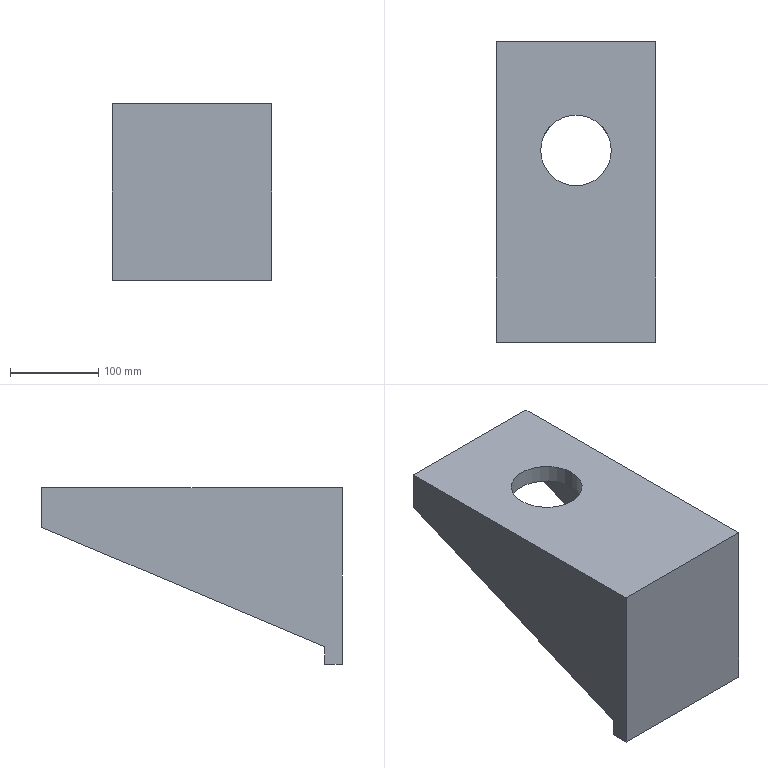Component | SolidWorks | CylinderBaseBaffle-1 | 1 solid | 14 faces | box 180 x 340 x 200 mm | volume 2955469 mm3 | plane 12 | cylinder 2 | commonest cylinder face diameters 80 x2
build123d program:
from build123d import *

# Parameters (mm, degrees)
SKETCH1_W           = 180
SKETCH1_H           = 320
BOSS_EXTRUDE1_DEPTH = 20
SKETCH2_W           = 180
SKETCH2_H           = 200
BOSS_EXTRUDE2_DEPTH = 20
BOSS_EXTRUDE3_DEPTH = 20
SKETCH5_R           = 40
CUT_EXTRUDE2_DEPTH  = 50


with BuildPart() as part:
    # Sketch1 → Boss-Extrude1 (new body)
    with BuildSketch(Plane.XY):
        Rectangle(SKETCH1_W, SKETCH1_H)
    extrude(amount=BOSS_EXTRUDE1_DEPTH)

    # Sketch2 → Boss-Extrude2 (add)
    with BuildSketch(Plane.XZ.offset(160)):
        with Locations((0, -80)):
            Rectangle(SKETCH2_W, SKETCH2_H)
    extrude(amount=BOSS_EXTRUDE2_DEPTH)

    # Sketch3 → Boss-Extrude3 (add)
    with BuildSketch(Plane(origin=(90, 0, 0), x_dir=(0, 0, -1), z_dir=(1, 0, 0))):
        Polygon((0, 160), (25, 160), (160, -160), (0, -160), align=None)
    boss_extrude3 = extrude(amount=-BOSS_EXTRUDE3_DEPTH)

    # Mirror1: Boss-Extrude3 across plane
    add(boss_extrude3.mirror(Plane(origin=(0, 0, 0), x_dir=(0, 0, 1), z_dir=(1, 0, 0))))

    # Sketch5 → Cut-Extrude2 (cut)
    with BuildSketch(Plane(origin=(0, 0, 0), x_dir=(-1, 0, 0), z_dir=(0, 0, -1))):
        with Locations((0, 36.859)):
            Circle(SKETCH5_R)
    extrude(amount=-CUT_EXTRUDE2_DEPTH, mode=Mode.SUBTRACT)


solid = part.part

# Placed as in the assembly
solid = solid.moved(Location((-7.456, -34.275, 560), (0, 0, 0)))
STEP:
#1=COLOUR_RGB('',0.7922,0.8196,0.9333);
#2=FILL_AREA_STYLE_COLOUR('',#1);
#3=FILL_AREA_STYLE('',(#2));
#4=SURFACE_STYLE_FILL_AREA(#3);
#5=SURFACE_SIDE_STYLE('',(#4));
#6=SURFACE_STYLE_USAGE(.BOTH.,#5);
#7=PRESENTATION_STYLE_ASSIGNMENT((#6));
#8=CARTESIAN_POINT('',(-1.868,0.1017,22.835));
#9=VERTEX_POINT('',#8);
#10=CARTESIAN_POINT('',(1.281,0.1017,22.835));
#11=VERTEX_POINT('',#10);
#12=CARTESIAN_POINT('',(-0.2935,0.1017,22.835));
#13=DIRECTION('',(0.,0.,1.));
#14=DIRECTION('',(1.,0.,0.));
#15=AXIS2_PLACEMENT_3D('',#12,#13,#14);
#16=CIRCLE('',#15,1.575);
#17=EDGE_CURVE('',#9,#11,#16,.T.);
#18=ORIENTED_EDGE('',*,*,#17,.T.);
#19=CARTESIAN_POINT('',(1.281,0.1017,22.047));
#20=VERTEX_POINT('',#19);
#21=CARTESIAN_POINT('',(1.281,0.1017,24.016));
#22=DIRECTION('',(0.,0.,-1.));
#23=VECTOR('',#22,39.37);
#24=LINE('',#21,#23);
#25=EDGE_CURVE('',#11,#20,#24,.T.);
#26=ORIENTED_EDGE('',*,*,#25,.T.);
#27=CARTESIAN_POINT('',(-1.868,0.1017,22.047));
#28=VERTEX_POINT('',#27);
#29=CARTESIAN_POINT('',(-0.2935,0.1017,22.047));
#30=DIRECTION('',(0.,0.,-1.));
#31=DIRECTION('',(-1.,0.,0.));
#32=AXIS2_PLACEMENT_3D('',#29,#30,#31);
#33=CIRCLE('',#32,1.575);
#34=EDGE_CURVE('',#20,#28,#33,.T.);
#35=ORIENTED_EDGE('',*,*,#34,.T.);
#36=CARTESIAN_POINT('',(-1.868,0.1017,24.016));
#37=DIRECTION('',(0.,0.,-1.));
#38=VECTOR('',#37,39.37);
#39=LINE('',#36,#38);
#40=EDGE_CURVE('',#9,#28,#39,.T.);
#41=ORIENTED_EDGE('',*,*,#40,.F.);
#42=EDGE_LOOP('',(#18,#26,#35,#41));
#43=FACE_OUTER_BOUND('',#42,.T.);
#44=CARTESIAN_POINT('',(-0.2935,0.1017,24.016));
#45=DIRECTION('',(0.,0.,-1.));
#46=DIRECTION('',(-1.,0.,0.));
#47=AXIS2_PLACEMENT_3D('',#44,#45,#46);
#48=CYLINDRICAL_SURFACE('',#47,1.575);
#49=ADVANCED_FACE('',(#43),#48,.F.);
#50=CARTESIAN_POINT('',(-3.049,-7.649,15.748));
#51=VERTEX_POINT('',#50);
#52=CARTESIAN_POINT('',(-3.837,-7.649,15.748));
#53=VERTEX_POINT('',#52);
#54=CARTESIAN_POINT('',(-3.049,-7.649,15.748));
#55=DIRECTION('',(-1.,0.,0.));
#56=VECTOR('',#55,39.37);
#57=LINE('',#54,#56);
#58=EDGE_CURVE('',#51,#53,#57,.T.);
#59=ORIENTED_EDGE('',*,*,#58,.F.);
#60=CARTESIAN_POINT('',(-3.049,-7.649,22.047));
#61=VERTEX_POINT('',#60);
#62=CARTESIAN_POINT('',(-3.049,-7.649,15.748));
#63=DIRECTION('',(0.,0.,-1.));
#64=VECTOR('',#63,39.37);
#65=LINE('',#62,#64);
#66=EDGE_CURVE('',#61,#51,#65,.T.);
#67=ORIENTED_EDGE('',*,*,#66,.F.);
#68=CARTESIAN_POINT('',(2.462,-7.649,22.047));
#69=VERTEX_POINT('',#68);
#70=CARTESIAN_POINT('',(3.25,-7.649,22.047));
#71=DIRECTION('',(1.,0.,0.));
#72=VECTOR('',#71,39.37);
#73=LINE('',#70,#72);
#74=EDGE_CURVE('',#61,#69,#73,.T.);
#75=ORIENTED_EDGE('',*,*,#74,.T.);
#76=CARTESIAN_POINT('',(2.462,-7.649,15.748));
#77=VERTEX_POINT('',#76);
#78=CARTESIAN_POINT('',(2.462,-7.649,15.748));
#79=DIRECTION('',(0.,0.,-1.));
#80=VECTOR('',#79,39.37);
#81=LINE('',#78,#80);
#82=EDGE_CURVE('',#69,#77,#81,.T.);
#83=ORIENTED_EDGE('',*,*,#82,.T.);
#84=CARTESIAN_POINT('',(3.25,-7.649,15.748));
#85=VERTEX_POINT('',#84);
#86=CARTESIAN_POINT('',(2.462,-7.649,15.748));
#87=DIRECTION('',(1.,0.,0.));
#88=VECTOR('',#87,39.37);
#89=LINE('',#86,#88);
#90=EDGE_CURVE('',#77,#85,#89,.T.);
#91=ORIENTED_EDGE('',*,*,#90,.T.);
#92=CARTESIAN_POINT('',(3.25,-7.649,14.961));
#93=VERTEX_POINT('',#92);
#94=CARTESIAN_POINT('',(3.25,-7.649,22.835));
#95=DIRECTION('',(-0.,0.,1.));
#96=VECTOR('',#95,39.37);
#97=LINE('',#94,#96);
#98=EDGE_CURVE('',#93,#85,#97,.T.);
#99=ORIENTED_EDGE('',*,*,#98,.F.);
#100=CARTESIAN_POINT('',(-3.837,-7.649,14.961));
#101=VERTEX_POINT('',#100);
#102=CARTESIAN_POINT('',(-3.837,-7.649,14.961));
#103=DIRECTION('',(1.,0.,0.));
#104=VECTOR('',#103,39.37);
#105=LINE('',#102,#104);
#106=EDGE_CURVE('',#101,#93,#105,.T.);
#107=ORIENTED_EDGE('',*,*,#106,.F.);
#108=CARTESIAN_POINT('',(-3.837,-7.649,22.835));
#109=DIRECTION('',(0.,0.,-1.));
#110=VECTOR('',#109,39.37);
#111=LINE('',#108,#110);
#112=EDGE_CURVE('',#53,#101,#111,.T.);
#113=ORIENTED_EDGE('',*,*,#112,.F.);
#114=EDGE_LOOP('',(#59,#67,#75,#83,#91,#99,#107,#113));
#115=FACE_OUTER_BOUND('',#114,.T.);
#116=CARTESIAN_POINT('',(-3.837,-7.649,14.961));
#117=DIRECTION('',(0.,-1.,0.));
#118=DIRECTION('',(0.,0.,-1.));
#119=AXIS2_PLACEMENT_3D('',#116,#117,#118);
#120=PLANE('',#119);
#121=ADVANCED_FACE('',(#115),#120,.F.);
#122=CARTESIAN_POINT('',(-3.837,4.95,22.835));
#123=VERTEX_POINT('',#122);
#124=CARTESIAN_POINT('',(-3.837,4.95,21.063));
#125=VERTEX_POINT('',#124);
#126=CARTESIAN_POINT('',(-3.837,4.95,22.835));
#127=DIRECTION('',(0.,0.,-1.));
#128=VECTOR('',#127,39.37);
#129=LINE('',#126,#128);
#130=EDGE_CURVE('',#123,#125,#129,.T.);
#131=ORIENTED_EDGE('',*,*,#130,.T.);
#132=CARTESIAN_POINT('',(-3.837,4.95,21.063));
#133=DIRECTION('',(0.,0.9214,0.3887));
#134=VECTOR('',#133,39.37);
#135=LINE('',#132,#134);
#136=EDGE_CURVE('',#53,#125,#135,.T.);
#137=ORIENTED_EDGE('',*,*,#136,.F.);
#138=ORIENTED_EDGE('',*,*,#112,.T.);
#139=CARTESIAN_POINT('',(-3.837,-8.436,14.961));
#140=VERTEX_POINT('',#139);
#141=CARTESIAN_POINT('',(-3.837,-8.436,14.961));
#142=DIRECTION('',(0.,1.,0.));
#143=VECTOR('',#142,39.37);
#144=LINE('',#141,#143);
#145=EDGE_CURVE('',#140,#101,#144,.T.);
#146=ORIENTED_EDGE('',*,*,#145,.F.);
#147=CARTESIAN_POINT('',(-3.837,-8.436,22.835));
#148=VERTEX_POINT('',#147);
#149=CARTESIAN_POINT('',(-3.837,-8.436,22.835));
#150=DIRECTION('',(0.,0.,-1.));
#151=VECTOR('',#150,39.37);
#152=LINE('',#149,#151);
#153=EDGE_CURVE('',#148,#140,#152,.T.);
#154=ORIENTED_EDGE('',*,*,#153,.F.);
#155=CARTESIAN_POINT('',(-3.837,-7.649,22.835));
#156=DIRECTION('',(0.,-1.,0.));
#157=VECTOR('',#156,39.37);
#158=LINE('',#155,#157);
#159=EDGE_CURVE('',#123,#148,#158,.T.);
#160=ORIENTED_EDGE('',*,*,#159,.F.);
#161=EDGE_LOOP('',(#131,#137,#138,#146,#154,#160));
#162=FACE_OUTER_BOUND('',#161,.T.);
#163=CARTESIAN_POINT('',(-3.837,-7.649,22.835));
#164=DIRECTION('',(1.,0.,0.));
#165=DIRECTION('',(0.,0.,-1.));
#166=AXIS2_PLACEMENT_3D('',#163,#164,#165);
#167=PLANE('',#166);
#168=ADVANCED_FACE('',(#162),#167,.F.);
#169=CARTESIAN_POINT('',(3.25,4.95,21.063));
#170=VERTEX_POINT('',#169);
#171=CARTESIAN_POINT('',(3.25,4.95,21.063));
#172=DIRECTION('',(0.,0.9214,0.3887));
#173=VECTOR('',#172,39.37);
#174=LINE('',#171,#173);
#175=EDGE_CURVE('',#85,#170,#174,.T.);
#176=ORIENTED_EDGE('',*,*,#175,.T.);
#177=CARTESIAN_POINT('',(3.25,4.95,22.835));
#178=VERTEX_POINT('',#177);
#179=CARTESIAN_POINT('',(3.25,4.95,22.835));
#180=DIRECTION('',(0.,0.,-1.));
#181=VECTOR('',#180,39.37);
#182=LINE('',#179,#181);
#183=EDGE_CURVE('',#178,#170,#182,.T.);
#184=ORIENTED_EDGE('',*,*,#183,.F.);
#185=CARTESIAN_POINT('',(3.25,-8.436,22.835));
#186=VERTEX_POINT('',#185);
#187=CARTESIAN_POINT('',(3.25,-7.649,22.835));
#188=DIRECTION('',(0.,1.,0.));
#189=VECTOR('',#188,39.37);
#190=LINE('',#187,#189);
#191=EDGE_CURVE('',#186,#178,#190,.T.);
#192=ORIENTED_EDGE('',*,*,#191,.F.);
#193=CARTESIAN_POINT('',(3.25,-8.436,14.961));
#194=VERTEX_POINT('',#193);
#195=CARTESIAN_POINT('',(3.25,-8.436,22.835));
#196=DIRECTION('',(-0.,0.,1.));
#197=VECTOR('',#196,39.37);
#198=LINE('',#195,#197);
#199=EDGE_CURVE('',#194,#186,#198,.T.);
#200=ORIENTED_EDGE('',*,*,#199,.F.);
#201=CARTESIAN_POINT('',(3.25,-8.436,14.961));
#202=DIRECTION('',(0.,1.,0.));
#203=VECTOR('',#202,39.37);
#204=LINE('',#201,#203);
#205=EDGE_CURVE('',#194,#93,#204,.T.);
#206=ORIENTED_EDGE('',*,*,#205,.T.);
#207=ORIENTED_EDGE('',*,*,#98,.T.);
#208=EDGE_LOOP('',(#176,#184,#192,#200,#206,#207));
#209=FACE_OUTER_BOUND('',#208,.T.);
#210=CARTESIAN_POINT('',(3.25,-7.649,22.835));
#211=DIRECTION('',(-1.,0.,0.));
#212=DIRECTION('',(0.,0.,1.));
#213=AXIS2_PLACEMENT_3D('',#210,#211,#212);
#214=PLANE('',#213);
#215=ADVANCED_FACE('',(#209),#214,.F.);
#216=ORIENTED_EDGE('',*,*,#183,.T.);
#217=CARTESIAN_POINT('',(2.462,4.95,21.063));
#218=VERTEX_POINT('',#217);
#219=CARTESIAN_POINT('',(2.462,4.95,21.063));
#220=DIRECTION('',(1.,0.,0.));
#221=VECTOR('',#220,39.37);
#222=LINE('',#219,#221);
#223=EDGE_CURVE('',#218,#170,#222,.T.);
#224=ORIENTED_EDGE('',*,*,#223,.F.);
#225=CARTESIAN_POINT('',(2.462,4.95,22.047));
#226=VERTEX_POINT('',#225);
#227=CARTESIAN_POINT('',(2.462,4.95,22.047));
#228=DIRECTION('',(0.,0.,1.));
#229=VECTOR('',#228,39.37);
#230=LINE('',#227,#229);
#231=EDGE_CURVE('',#218,#226,#230,.T.);
#232=ORIENTED_EDGE('',*,*,#231,.T.);
#233=CARTESIAN_POINT('',(-3.049,4.95,22.047));
#234=VERTEX_POINT('',#233);
#235=CARTESIAN_POINT('',(3.25,4.95,22.047));
#236=DIRECTION('',(-1.,0.,0.));
#237=VECTOR('',#236,39.37);
#238=LINE('',#235,#237);
#239=EDGE_CURVE('',#226,#234,#238,.T.);
#240=ORIENTED_EDGE('',*,*,#239,.T.);
#241=CARTESIAN_POINT('',(-3.049,4.95,21.063));
#242=VERTEX_POINT('',#241);
#243=CARTESIAN_POINT('',(-3.049,4.95,22.047));
#244=DIRECTION('',(0.,0.,1.));
#245=VECTOR('',#244,39.37);
#246=LINE('',#243,#245);
#247=EDGE_CURVE('',#242,#234,#246,.T.);
#248=ORIENTED_EDGE('',*,*,#247,.F.);
#249=CARTESIAN_POINT('',(-3.049,4.95,21.063));
#250=DIRECTION('',(-1.,0.,0.));
#251=VECTOR('',#250,39.37);
#252=LINE('',#249,#251);
#253=EDGE_CURVE('',#242,#125,#252,.T.);
#254=ORIENTED_EDGE('',*,*,#253,.T.);
#255=ORIENTED_EDGE('',*,*,#130,.F.);
#256=CARTESIAN_POINT('',(3.25,4.95,22.835));
#257=DIRECTION('',(-1.,0.,0.));
#258=VECTOR('',#257,39.37);
#259=LINE('',#256,#258);
#260=EDGE_CURVE('',#178,#123,#259,.T.);
#261=ORIENTED_EDGE('',*,*,#260,.F.);
#262=EDGE_LOOP('',(#216,#224,#232,#240,#248,#254,#255,#261));
#263=FACE_OUTER_BOUND('',#262,.T.);
#264=CARTESIAN_POINT('',(3.25,4.95,22.835));
#265=DIRECTION('',(0.,-1.,0.));
#266=DIRECTION('',(0.,0.,-1.));
#267=AXIS2_PLACEMENT_3D('',#264,#265,#266);
#268=PLANE('',#267);
#269=ADVANCED_FACE('',(#263),#268,.F.);
#270=ORIENTED_EDGE('',*,*,#17,.F.);
#271=CARTESIAN_POINT('',(-0.2935,0.1017,22.835));
#272=DIRECTION('',(0.,0.,1.));
#273=DIRECTION('',(1.,0.,0.));
#274=AXIS2_PLACEMENT_3D('',#271,#272,#273);
#275=CIRCLE('',#274,1.575);
#276=EDGE_CURVE('',#11,#9,#275,.T.);
#277=ORIENTED_EDGE('',*,*,#276,.F.);
#278=EDGE_LOOP('',(#270,#277));
#279=FACE_BOUND('',#278,.T.);
#280=ORIENTED_EDGE('',*,*,#159,.T.);
#281=CARTESIAN_POINT('',(-3.837,-8.436,22.835));
#282=DIRECTION('',(-1.,0.,0.));
#283=VECTOR('',#282,39.37);
#284=LINE('',#281,#283);
#285=EDGE_CURVE('',#186,#148,#284,.T.);
#286=ORIENTED_EDGE('',*,*,#285,.F.);
#287=ORIENTED_EDGE('',*,*,#191,.T.);
#288=ORIENTED_EDGE('',*,*,#260,.T.);
#289=EDGE_LOOP('',(#280,#286,#287,#288));
#290=FACE_OUTER_BOUND('',#289,.T.);
#291=CARTESIAN_POINT('',(-3.837,4.95,22.835));
#292=DIRECTION('',(0.,0.,1.));
#293=DIRECTION('',(1.,0.,0.));
#294=AXIS2_PLACEMENT_3D('',#291,#292,#293);
#295=PLANE('',#294);
#296=ADVANCED_FACE('',(#279,#290),#295,.T.);
#297=CARTESIAN_POINT('',(-0.2935,0.1017,22.047));
#298=DIRECTION('',(0.,0.,-1.));
#299=DIRECTION('',(-1.,0.,0.));
#300=AXIS2_PLACEMENT_3D('',#297,#298,#299);
#301=CIRCLE('',#300,1.575);
#302=EDGE_CURVE('',#28,#20,#301,.T.);
#303=ORIENTED_EDGE('',*,*,#302,.F.);
#304=ORIENTED_EDGE('',*,*,#34,.F.);
#305=EDGE_LOOP('',(#303,#304));
#306=FACE_BOUND('',#305,.T.);
#307=ORIENTED_EDGE('',*,*,#74,.F.);
#308=CARTESIAN_POINT('',(-3.049,-7.649,22.047));
#309=DIRECTION('',(0.,-1.,0.));
#310=VECTOR('',#309,39.37);
#311=LINE('',#308,#310);
#312=EDGE_CURVE('',#234,#61,#311,.T.);
#313=ORIENTED_EDGE('',*,*,#312,.F.);
#314=ORIENTED_EDGE('',*,*,#239,.F.);
#315=CARTESIAN_POINT('',(2.462,-7.649,22.047));
#316=DIRECTION('',(0.,-1.,0.));
#317=VECTOR('',#316,39.37);
#318=LINE('',#315,#317);
#319=EDGE_CURVE('',#226,#69,#318,.T.);
#320=ORIENTED_EDGE('',*,*,#319,.T.);
#321=EDGE_LOOP('',(#307,#313,#314,#320));
#322=FACE_OUTER_BOUND('',#321,.T.);
#323=CARTESIAN_POINT('',(-3.837,4.95,22.047));
#324=DIRECTION('',(0.,0.,1.));
#325=DIRECTION('',(1.,0.,0.));
#326=AXIS2_PLACEMENT_3D('',#323,#324,#325);
#327=PLANE('',#326);
#328=ADVANCED_FACE('',(#306,#322),#327,.F.);
#329=ORIENTED_EDGE('',*,*,#106,.T.);
#330=ORIENTED_EDGE('',*,*,#205,.F.);
#331=CARTESIAN_POINT('',(-3.837,-8.436,14.961));
#332=DIRECTION('',(1.,0.,0.));
#333=VECTOR('',#332,39.37);
#334=LINE('',#331,#333);
#335=EDGE_CURVE('',#140,#194,#334,.T.);
#336=ORIENTED_EDGE('',*,*,#335,.F.);
#337=ORIENTED_EDGE('',*,*,#145,.T.);
#338=EDGE_LOOP('',(#329,#330,#336,#337));
#339=FACE_OUTER_BOUND('',#338,.T.);
#340=CARTESIAN_POINT('',(-3.837,-8.436,14.961));
#341=DIRECTION('',(0.,0.,1.));
#342=DIRECTION('',(1.,0.,0.));
#343=AXIS2_PLACEMENT_3D('',#340,#341,#342);
#344=PLANE('',#343);
#345=ADVANCED_FACE('',(#339),#344,.F.);
#346=ORIENTED_EDGE('',*,*,#153,.T.);
#347=ORIENTED_EDGE('',*,*,#335,.T.);
#348=ORIENTED_EDGE('',*,*,#199,.T.);
#349=ORIENTED_EDGE('',*,*,#285,.T.);
#350=EDGE_LOOP('',(#346,#347,#348,#349));
#351=FACE_OUTER_BOUND('',#350,.T.);
#352=CARTESIAN_POINT('',(-3.837,-8.436,14.961));
#353=DIRECTION('',(0.,-1.,0.));
#354=DIRECTION('',(0.,0.,-1.));
#355=AXIS2_PLACEMENT_3D('',#352,#353,#354);
#356=PLANE('',#355);
#357=ADVANCED_FACE('',(#351),#356,.T.);
#358=ORIENTED_EDGE('',*,*,#175,.F.);
#359=ORIENTED_EDGE('',*,*,#90,.F.);
#360=CARTESIAN_POINT('',(2.462,4.95,21.063));
#361=DIRECTION('',(0.,0.9214,0.3887));
#362=VECTOR('',#361,39.37);
#363=LINE('',#360,#362);
#364=EDGE_CURVE('',#77,#218,#363,.T.);
#365=ORIENTED_EDGE('',*,*,#364,.T.);
#366=ORIENTED_EDGE('',*,*,#223,.T.);
#367=EDGE_LOOP('',(#358,#359,#365,#366));
#368=FACE_OUTER_BOUND('',#367,.T.);
#369=CARTESIAN_POINT('',(2.462,4.95,21.063));
#370=DIRECTION('',(0.,0.3887,-0.9214));
#371=DIRECTION('',(0.,0.9214,0.3887));
#372=AXIS2_PLACEMENT_3D('',#369,#370,#371);
#373=PLANE('',#372);
#374=ADVANCED_FACE('',(#368),#373,.T.);
#375=ORIENTED_EDGE('',*,*,#319,.F.);
#376=ORIENTED_EDGE('',*,*,#231,.F.);
#377=ORIENTED_EDGE('',*,*,#364,.F.);
#378=ORIENTED_EDGE('',*,*,#82,.F.);
#379=EDGE_LOOP('',(#375,#376,#377,#378));
#380=FACE_OUTER_BOUND('',#379,.T.);
#381=CARTESIAN_POINT('',(2.462,4.95,22.047));
#382=DIRECTION('',(-1.,0.,0.));
#383=DIRECTION('',(0.,0.,1.));
#384=AXIS2_PLACEMENT_3D('',#381,#382,#383);
#385=PLANE('',#384);
#386=ADVANCED_FACE('',(#380),#385,.T.);
#387=ORIENTED_EDGE('',*,*,#136,.T.);
#388=ORIENTED_EDGE('',*,*,#253,.F.);
#389=CARTESIAN_POINT('',(-3.049,4.95,21.063));
#390=DIRECTION('',(0.,0.9214,0.3887));
#391=VECTOR('',#390,39.37);
#392=LINE('',#389,#391);
#393=EDGE_CURVE('',#51,#242,#392,.T.);
#394=ORIENTED_EDGE('',*,*,#393,.F.);
#395=ORIENTED_EDGE('',*,*,#58,.T.);
#396=EDGE_LOOP('',(#387,#388,#394,#395));
#397=FACE_OUTER_BOUND('',#396,.T.);
#398=CARTESIAN_POINT('',(-3.049,4.95,21.063));
#399=DIRECTION('',(0.,-0.3887,0.9214));
#400=DIRECTION('',(0.,-0.9214,-0.3887));
#401=AXIS2_PLACEMENT_3D('',#398,#399,#400);
#402=PLANE('',#401);
#403=ADVANCED_FACE('',(#397),#402,.F.);
#404=ORIENTED_EDGE('',*,*,#312,.T.);
#405=ORIENTED_EDGE('',*,*,#66,.T.);
#406=ORIENTED_EDGE('',*,*,#393,.T.);
#407=ORIENTED_EDGE('',*,*,#247,.T.);
#408=EDGE_LOOP('',(#404,#405,#406,#407));
#409=FACE_OUTER_BOUND('',#408,.T.);
#410=CARTESIAN_POINT('',(-3.049,4.95,22.047));
#411=DIRECTION('',(1.,0.,0.));
#412=DIRECTION('',(0.,0.,1.));
#413=AXIS2_PLACEMENT_3D('',#410,#411,#412);
#414=PLANE('',#413);
#415=ADVANCED_FACE('',(#409),#414,.T.);
#416=ORIENTED_EDGE('',*,*,#25,.F.);
#417=ORIENTED_EDGE('',*,*,#276,.T.);
#418=ORIENTED_EDGE('',*,*,#40,.T.);
#419=ORIENTED_EDGE('',*,*,#302,.T.);
#420=EDGE_LOOP('',(#416,#417,#418,#419));
#421=FACE_OUTER_BOUND('',#420,.T.);
#422=CARTESIAN_POINT('',(-0.2935,0.1017,24.016));
#423=DIRECTION('',(0.,0.,-1.));
#424=DIRECTION('',(-1.,0.,0.));
#425=AXIS2_PLACEMENT_3D('',#422,#423,#424);
#426=CYLINDRICAL_SURFACE('',#425,1.575);
#427=ADVANCED_FACE('',(#421),#426,.F.);
#428=CLOSED_SHELL('',(#49,#121,#168,#215,#269,#296,#328,#345,#357,#374,#386,#403,#415,#427));
#429=MANIFOLD_SOLID_BREP('',#428);
#430=STYLED_ITEM('',(#7),#429);
#431=PRESENTATION_LAYER_ASSIGNMENT('','',(#430));
#432=(LENGTH_UNIT()NAMED_UNIT(*)SI_UNIT($,.METRE.));
#433=LENGTH_MEASURE_WITH_UNIT(LENGTH_MEASURE(0.0254),#432);
#434=DIMENSIONAL_EXPONENTS(1.,0.,0.,0.,0.,0.,0.);
#435=(CONVERSION_BASED_UNIT('',#433)LENGTH_UNIT()NAMED_UNIT(#434));
#436=UNCERTAINTY_MEASURE_WITH_UNIT(LENGTH_MEASURE(0.00001),#435,'','');
#437=(NAMED_UNIT(*)PLANE_ANGLE_UNIT()SI_UNIT($,.RADIAN.));
#438=(NAMED_UNIT(*)SI_UNIT($,.STERADIAN.)SOLID_ANGLE_UNIT());
#439=(GEOMETRIC_REPRESENTATION_CONTEXT(3)GLOBAL_UNCERTAINTY_ASSIGNED_CONTEXT((#436))GLOBAL_UNIT_ASSIGNED_CONTEXT((#435,#437,#438))REPRESENTATION_CONTEXT('',''));
#440=MECHANICAL_DESIGN_GEOMETRIC_PRESENTATION_REPRESENTATION('',(#430),#439);
#441=CARTESIAN_POINT('',(0.,0.,0.));
#442=DIRECTION('',(0.,0.,1.));
#443=DIRECTION('',(1.,0.,0.));
#444=AXIS2_PLACEMENT_3D('',#441,#442,#443);
#445=(LENGTH_UNIT()NAMED_UNIT(*)SI_UNIT($,.METRE.));
#446=LENGTH_MEASURE_WITH_UNIT(LENGTH_MEASURE(0.0254),#445);
#447=DIMENSIONAL_EXPONENTS(1.,0.,0.,0.,0.,0.,0.);
#448=(CONVERSION_BASED_UNIT('',#446)LENGTH_UNIT()NAMED_UNIT(#447));
#449=UNCERTAINTY_MEASURE_WITH_UNIT(LENGTH_MEASURE(0.00001),#448,'','');
#450=(NAMED_UNIT(*)PLANE_ANGLE_UNIT()SI_UNIT($,.RADIAN.));
#451=(NAMED_UNIT(*)SI_UNIT($,.STERADIAN.)SOLID_ANGLE_UNIT());
#452=(GEOMETRIC_REPRESENTATION_CONTEXT(3)GLOBAL_UNCERTAINTY_ASSIGNED_CONTEXT((#449))GLOBAL_UNIT_ASSIGNED_CONTEXT((#448,#450,#451))REPRESENTATION_CONTEXT('',''));
#453=ADVANCED_BREP_SHAPE_REPRESENTATION('',(#429,#444),#452);